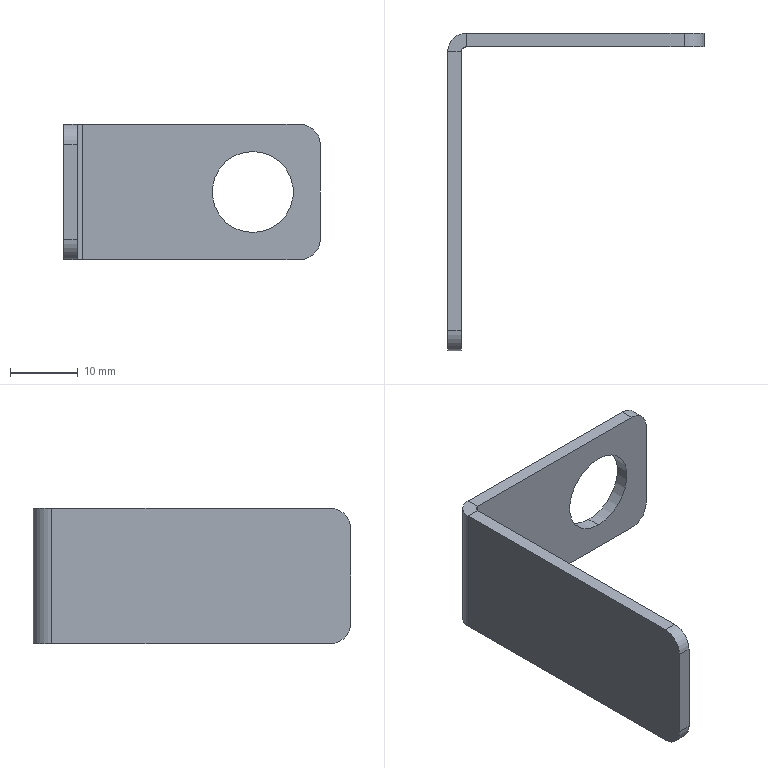Component | SolidWorks | CHEN123-AA-20-1 | 1 solid | 20 faces | box 38 x 47 x 20 mm | volume 3049 mm3 | plane 12 | cylinder 8 | commonest cylinder face diameters 6 x4 12 x2 1.473 x1 5.473 x1
STEP:
#1=CARTESIAN_POINT('',(-0.07876,2.126,-15.984));
#2=VERTEX_POINT('',#1);
#3=CARTESIAN_POINT('',(-0.07876,2.126,-15.512));
#4=VERTEX_POINT('',#3);
#5=CARTESIAN_POINT('',(-0.07876,2.126,-15.748));
#6=DIRECTION('',(-0.,-1.,0.));
#7=DIRECTION('',(-1.,0.,0.));
#8=AXIS2_PLACEMENT_3D('',#5,#6,#7);
#9=CIRCLE('',#8,0.2362);
#10=EDGE_CURVE('',#2,#4,#9,.T.);
#11=ORIENTED_EDGE('',*,*,#10,.T.);
#12=CARTESIAN_POINT('',(-0.07876,2.205,-15.512));
#13=VERTEX_POINT('',#12);
#14=CARTESIAN_POINT('',(-0.07876,2.205,-15.512));
#15=DIRECTION('',(0.,1.,-0.));
#16=VECTOR('',#15,39.37);
#17=LINE('',#14,#16);
#18=EDGE_CURVE('',#4,#13,#17,.T.);
#19=ORIENTED_EDGE('',*,*,#18,.T.);
#20=CARTESIAN_POINT('',(-0.07876,2.205,-15.984));
#21=VERTEX_POINT('',#20);
#22=CARTESIAN_POINT('',(-0.07876,2.205,-15.748));
#23=DIRECTION('',(0.,1.,-0.));
#24=DIRECTION('',(0.,0.,-1.));
#25=AXIS2_PLACEMENT_3D('',#22,#23,#24);
#26=CIRCLE('',#25,0.2362);
#27=EDGE_CURVE('',#13,#21,#26,.T.);
#28=ORIENTED_EDGE('',*,*,#27,.T.);
#29=CARTESIAN_POINT('',(-0.07876,2.205,-15.984));
#30=DIRECTION('',(0.,1.,-0.));
#31=VECTOR('',#30,39.37);
#32=LINE('',#29,#31);
#33=EDGE_CURVE('',#2,#21,#32,.T.);
#34=ORIENTED_EDGE('',*,*,#33,.F.);
#35=EDGE_LOOP('',(#11,#19,#28,#34));
#36=FACE_OUTER_BOUND('',#35,.T.);
#37=CARTESIAN_POINT('',(-0.07876,2.205,-15.748));
#38=DIRECTION('',(0.,1.,-0.));
#39=DIRECTION('',(0.,0.,-1.));
#40=AXIS2_PLACEMENT_3D('',#37,#38,#39);
#41=CYLINDRICAL_SURFACE('',#40,0.2362);
#42=ADVANCED_FACE('',(#36),#41,.F.);
#43=CARTESIAN_POINT('',(-1.073,2.126,-16.142));
#44=VERTEX_POINT('',#43);
#45=CARTESIAN_POINT('',(-1.073,2.205,-16.142));
#46=VERTEX_POINT('',#45);
#47=CARTESIAN_POINT('',(-1.073,2.126,-16.142));
#48=DIRECTION('',(0.,1.,-0.));
#49=VECTOR('',#48,39.37);
#50=LINE('',#47,#49);
#51=EDGE_CURVE('',#44,#46,#50,.T.);
#52=ORIENTED_EDGE('',*,*,#51,.F.);
#53=CARTESIAN_POINT('',(-1.102,2.097,-16.142));
#54=VERTEX_POINT('',#53);
#55=CARTESIAN_POINT('',(-1.073,2.097,-16.142));
#56=DIRECTION('',(0.,-0.,-1.));
#57=DIRECTION('',(1.,0.,0.));
#58=AXIS2_PLACEMENT_3D('',#55,#56,#57);
#59=CIRCLE('',#58,0.029);
#60=EDGE_CURVE('',#54,#44,#59,.T.);
#61=ORIENTED_EDGE('',*,*,#60,.F.);
#62=CARTESIAN_POINT('',(-1.181,2.097,-16.142));
#63=VERTEX_POINT('',#62);
#64=CARTESIAN_POINT('',(-1.181,2.097,-16.142));
#65=DIRECTION('',(1.,0.,-0.));
#66=VECTOR('',#65,39.37);
#67=LINE('',#64,#66);
#68=EDGE_CURVE('',#63,#54,#67,.T.);
#69=ORIENTED_EDGE('',*,*,#68,.F.);
#70=CARTESIAN_POINT('',(-1.073,2.097,-16.142));
#71=DIRECTION('',(0.,-0.,-1.));
#72=DIRECTION('',(-1.,0.,0.));
#73=AXIS2_PLACEMENT_3D('',#70,#71,#72);
#74=CIRCLE('',#73,0.1077);
#75=EDGE_CURVE('',#63,#46,#74,.T.);
#76=ORIENTED_EDGE('',*,*,#75,.T.);
#77=EDGE_LOOP('',(#52,#61,#69,#76));
#78=FACE_OUTER_BOUND('',#77,.T.);
#79=CARTESIAN_POINT('',(-1.073,2.126,-16.142));
#80=DIRECTION('',(0.,-0.,-1.));
#81=DIRECTION('',(-1.,0.,0.));
#82=AXIS2_PLACEMENT_3D('',#79,#80,#81);
#83=PLANE('',#82);
#84=ADVANCED_FACE('',(#78),#83,.T.);
#85=CARTESIAN_POINT('',(0.1968,2.205,-16.142));
#86=VERTEX_POINT('',#85);
#87=CARTESIAN_POINT('',(-1.102,2.205,-16.142));
#88=DIRECTION('',(1.,-0.,0.));
#89=VECTOR('',#88,39.37);
#90=LINE('',#87,#89);
#91=EDGE_CURVE('',#46,#86,#90,.T.);
#92=ORIENTED_EDGE('',*,*,#91,.T.);
#93=CARTESIAN_POINT('',(0.1968,2.126,-16.142));
#94=VERTEX_POINT('',#93);
#95=CARTESIAN_POINT('',(0.1968,2.097,-16.142));
#96=DIRECTION('',(0.,-1.,0.));
#97=VECTOR('',#96,39.37);
#98=LINE('',#95,#97);
#99=EDGE_CURVE('',#86,#94,#98,.T.);
#100=ORIENTED_EDGE('',*,*,#99,.T.);
#101=CARTESIAN_POINT('',(-1.102,2.126,-16.142));
#102=DIRECTION('',(1.,-0.,0.));
#103=VECTOR('',#102,39.37);
#104=LINE('',#101,#103);
#105=EDGE_CURVE('',#44,#94,#104,.T.);
#106=ORIENTED_EDGE('',*,*,#105,.F.);
#107=ORIENTED_EDGE('',*,*,#51,.T.);
#108=EDGE_LOOP('',(#92,#100,#106,#107));
#109=FACE_OUTER_BOUND('',#108,.T.);
#110=CARTESIAN_POINT('',(-1.181,2.097,-16.142));
#111=DIRECTION('',(0.,-0.,-1.));
#112=DIRECTION('',(-1.,0.,0.));
#113=AXIS2_PLACEMENT_3D('',#110,#111,#112);
#114=PLANE('',#113);
#115=ADVANCED_FACE('',(#109),#114,.T.);
#116=CARTESIAN_POINT('',(-1.102,2.097,-15.354));
#117=VERTEX_POINT('',#116);
#118=CARTESIAN_POINT('',(-1.181,2.097,-15.354));
#119=VERTEX_POINT('',#118);
#120=CARTESIAN_POINT('',(-1.102,2.097,-15.354));
#121=DIRECTION('',(-1.,-0.,0.));
#122=VECTOR('',#121,39.37);
#123=LINE('',#120,#122);
#124=EDGE_CURVE('',#117,#119,#123,.T.);
#125=ORIENTED_EDGE('',*,*,#124,.F.);
#126=CARTESIAN_POINT('',(-1.073,2.126,-15.354));
#127=VERTEX_POINT('',#126);
#128=CARTESIAN_POINT('',(-1.073,2.097,-15.354));
#129=DIRECTION('',(0.,-0.,-1.));
#130=DIRECTION('',(1.,0.,0.));
#131=AXIS2_PLACEMENT_3D('',#128,#129,#130);
#132=CIRCLE('',#131,0.029);
#133=EDGE_CURVE('',#117,#127,#132,.T.);
#134=ORIENTED_EDGE('',*,*,#133,.T.);
#135=CARTESIAN_POINT('',(-1.073,2.205,-15.354));
#136=VERTEX_POINT('',#135);
#137=CARTESIAN_POINT('',(-1.073,2.205,-15.354));
#138=DIRECTION('',(-0.,-1.,0.));
#139=VECTOR('',#138,39.37);
#140=LINE('',#137,#139);
#141=EDGE_CURVE('',#136,#127,#140,.T.);
#142=ORIENTED_EDGE('',*,*,#141,.F.);
#143=CARTESIAN_POINT('',(-1.073,2.097,-15.354));
#144=DIRECTION('',(0.,-0.,-1.));
#145=DIRECTION('',(-1.,0.,0.));
#146=AXIS2_PLACEMENT_3D('',#143,#144,#145);
#147=CIRCLE('',#146,0.1077);
#148=EDGE_CURVE('',#119,#136,#147,.T.);
#149=ORIENTED_EDGE('',*,*,#148,.F.);
#150=EDGE_LOOP('',(#125,#134,#142,#149));
#151=FACE_OUTER_BOUND('',#150,.T.);
#152=CARTESIAN_POINT('',(-1.102,2.097,-15.354));
#153=DIRECTION('',(0.,0.,1.));
#154=DIRECTION('',(1.,0.,0.));
#155=AXIS2_PLACEMENT_3D('',#152,#153,#154);
#156=PLANE('',#155);
#157=ADVANCED_FACE('',(#151),#156,.T.);
#158=CARTESIAN_POINT('',(-1.181,0.4725,-15.354));
#159=VERTEX_POINT('',#158);
#160=CARTESIAN_POINT('',(-1.181,0.3544,-15.354));
#161=DIRECTION('',(0.,1.,-0.));
#162=VECTOR('',#161,39.37);
#163=LINE('',#160,#162);
#164=EDGE_CURVE('',#159,#119,#163,.T.);
#165=ORIENTED_EDGE('',*,*,#164,.F.);
#166=CARTESIAN_POINT('',(-1.102,0.4725,-15.354));
#167=VERTEX_POINT('',#166);
#168=CARTESIAN_POINT('',(-1.073,0.4725,-15.354));
#169=DIRECTION('',(1.,0.,0.));
#170=VECTOR('',#169,39.37);
#171=LINE('',#168,#170);
#172=EDGE_CURVE('',#159,#167,#171,.T.);
#173=ORIENTED_EDGE('',*,*,#172,.T.);
#174=CARTESIAN_POINT('',(-1.102,0.3544,-15.354));
#175=DIRECTION('',(0.,1.,-0.));
#176=VECTOR('',#175,39.37);
#177=LINE('',#174,#176);
#178=EDGE_CURVE('',#167,#117,#177,.T.);
#179=ORIENTED_EDGE('',*,*,#178,.T.);
#180=ORIENTED_EDGE('',*,*,#124,.T.);
#181=EDGE_LOOP('',(#165,#173,#179,#180));
#182=FACE_OUTER_BOUND('',#181,.T.);
#183=CARTESIAN_POINT('',(-1.073,2.205,-15.354));
#184=DIRECTION('',(0.,0.,1.));
#185=DIRECTION('',(1.,0.,0.));
#186=AXIS2_PLACEMENT_3D('',#183,#184,#185);
#187=PLANE('',#186);
#188=ADVANCED_FACE('',(#182),#187,.T.);
#189=CARTESIAN_POINT('',(-0.07876,2.205,-15.748));
#190=DIRECTION('',(0.,1.,-0.));
#191=DIRECTION('',(0.,0.,-1.));
#192=AXIS2_PLACEMENT_3D('',#189,#190,#191);
#193=CIRCLE('',#192,0.2362);
#194=EDGE_CURVE('',#21,#13,#193,.T.);
#195=ORIENTED_EDGE('',*,*,#194,.F.);
#196=ORIENTED_EDGE('',*,*,#27,.F.);
#197=EDGE_LOOP('',(#195,#196));
#198=FACE_BOUND('',#197,.T.);
#199=CARTESIAN_POINT('',(0.1968,2.205,-15.354));
#200=VERTEX_POINT('',#199);
#201=CARTESIAN_POINT('',(-1.102,2.205,-15.354));
#202=DIRECTION('',(1.,-0.,0.));
#203=VECTOR('',#202,39.37);
#204=LINE('',#201,#203);
#205=EDGE_CURVE('',#136,#200,#204,.T.);
#206=ORIENTED_EDGE('',*,*,#205,.T.);
#207=CARTESIAN_POINT('',(0.3149,2.205,-15.472));
#208=VERTEX_POINT('',#207);
#209=CARTESIAN_POINT('',(0.1968,2.205,-15.472));
#210=DIRECTION('',(0.,1.,-0.));
#211=DIRECTION('',(-1.,0.,0.));
#212=AXIS2_PLACEMENT_3D('',#209,#210,#211);
#213=CIRCLE('',#212,0.1181);
#214=EDGE_CURVE('',#200,#208,#213,.T.);
#215=ORIENTED_EDGE('',*,*,#214,.T.);
#216=CARTESIAN_POINT('',(0.3149,2.205,-16.024));
#217=VERTEX_POINT('',#216);
#218=CARTESIAN_POINT('',(0.3149,2.205,-16.142));
#219=DIRECTION('',(0.,0.,1.));
#220=VECTOR('',#219,39.37);
#221=LINE('',#218,#220);
#222=EDGE_CURVE('',#217,#208,#221,.T.);
#223=ORIENTED_EDGE('',*,*,#222,.F.);
#224=CARTESIAN_POINT('',(0.1968,2.205,-16.024));
#225=DIRECTION('',(0.,1.,-0.));
#226=DIRECTION('',(-1.,0.,0.));
#227=AXIS2_PLACEMENT_3D('',#224,#225,#226);
#228=CIRCLE('',#227,0.1181);
#229=EDGE_CURVE('',#217,#86,#228,.T.);
#230=ORIENTED_EDGE('',*,*,#229,.T.);
#231=ORIENTED_EDGE('',*,*,#91,.F.);
#232=CARTESIAN_POINT('',(-1.073,2.205,-16.142));
#233=DIRECTION('',(0.,0.,1.));
#234=VECTOR('',#233,39.37);
#235=LINE('',#232,#234);
#236=EDGE_CURVE('',#46,#136,#235,.T.);
#237=ORIENTED_EDGE('',*,*,#236,.T.);
#238=EDGE_LOOP('',(#206,#215,#223,#230,#231,#237));
#239=FACE_OUTER_BOUND('',#238,.T.);
#240=CARTESIAN_POINT('',(-1.102,2.205,-16.142));
#241=DIRECTION('',(-0.,-1.,0.));
#242=DIRECTION('',(-1.,0.,-0.));
#243=AXIS2_PLACEMENT_3D('',#240,#241,#242);
#244=PLANE('',#243);
#245=ADVANCED_FACE('',(#198,#239),#244,.F.);
#246=ORIENTED_EDGE('',*,*,#222,.T.);
#247=CARTESIAN_POINT('',(0.3149,2.126,-15.472));
#248=VERTEX_POINT('',#247);
#249=CARTESIAN_POINT('',(0.3149,2.126,-15.472));
#250=DIRECTION('',(0.,-1.,0.));
#251=VECTOR('',#250,39.37);
#252=LINE('',#249,#251);
#253=EDGE_CURVE('',#208,#248,#252,.T.);
#254=ORIENTED_EDGE('',*,*,#253,.T.);
#255=CARTESIAN_POINT('',(0.3149,2.126,-16.024));
#256=VERTEX_POINT('',#255);
#257=CARTESIAN_POINT('',(0.3149,2.126,-16.142));
#258=DIRECTION('',(0.,0.,1.));
#259=VECTOR('',#258,39.37);
#260=LINE('',#257,#259);
#261=EDGE_CURVE('',#256,#248,#260,.T.);
#262=ORIENTED_EDGE('',*,*,#261,.F.);
#263=CARTESIAN_POINT('',(0.3149,2.126,-16.024));
#264=DIRECTION('',(0.,1.,-0.));
#265=VECTOR('',#264,39.37);
#266=LINE('',#263,#265);
#267=EDGE_CURVE('',#256,#217,#266,.T.);
#268=ORIENTED_EDGE('',*,*,#267,.T.);
#269=EDGE_LOOP('',(#246,#254,#262,#268));
#270=FACE_OUTER_BOUND('',#269,.T.);
#271=CARTESIAN_POINT('',(0.3149,2.126,-16.142));
#272=DIRECTION('',(1.,0.,0.));
#273=DIRECTION('',(0.,-0.,-1.));
#274=AXIS2_PLACEMENT_3D('',#271,#272,#273);
#275=PLANE('',#274);
#276=ADVANCED_FACE('',(#270),#275,.T.);
#277=ORIENTED_EDGE('',*,*,#10,.F.);
#278=CARTESIAN_POINT('',(-0.07876,2.126,-15.748));
#279=DIRECTION('',(-0.,-1.,0.));
#280=DIRECTION('',(-1.,0.,0.));
#281=AXIS2_PLACEMENT_3D('',#278,#279,#280);
#282=CIRCLE('',#281,0.2362);
#283=EDGE_CURVE('',#4,#2,#282,.T.);
#284=ORIENTED_EDGE('',*,*,#283,.F.);
#285=EDGE_LOOP('',(#277,#284));
#286=FACE_BOUND('',#285,.T.);
#287=ORIENTED_EDGE('',*,*,#261,.T.);
#288=CARTESIAN_POINT('',(0.1968,2.126,-15.354));
#289=VERTEX_POINT('',#288);
#290=CARTESIAN_POINT('',(0.1968,2.126,-15.472));
#291=DIRECTION('',(-0.,-1.,0.));
#292=DIRECTION('',(-1.,0.,0.));
#293=AXIS2_PLACEMENT_3D('',#290,#291,#292);
#294=CIRCLE('',#293,0.1181);
#295=EDGE_CURVE('',#248,#289,#294,.T.);
#296=ORIENTED_EDGE('',*,*,#295,.T.);
#297=CARTESIAN_POINT('',(-1.102,2.126,-15.354));
#298=DIRECTION('',(1.,-0.,0.));
#299=VECTOR('',#298,39.37);
#300=LINE('',#297,#299);
#301=EDGE_CURVE('',#127,#289,#300,.T.);
#302=ORIENTED_EDGE('',*,*,#301,.F.);
#303=CARTESIAN_POINT('',(-1.073,2.126,-16.142));
#304=DIRECTION('',(0.,0.,1.));
#305=VECTOR('',#304,39.37);
#306=LINE('',#303,#305);
#307=EDGE_CURVE('',#44,#127,#306,.T.);
#308=ORIENTED_EDGE('',*,*,#307,.F.);
#309=ORIENTED_EDGE('',*,*,#105,.T.);
#310=CARTESIAN_POINT('',(0.1968,2.126,-16.024));
#311=DIRECTION('',(-0.,-1.,0.));
#312=DIRECTION('',(-1.,0.,0.));
#313=AXIS2_PLACEMENT_3D('',#310,#311,#312);
#314=CIRCLE('',#313,0.1181);
#315=EDGE_CURVE('',#94,#256,#314,.T.);
#316=ORIENTED_EDGE('',*,*,#315,.T.);
#317=EDGE_LOOP('',(#287,#296,#302,#308,#309,#316));
#318=FACE_OUTER_BOUND('',#317,.T.);
#319=CARTESIAN_POINT('',(-1.102,2.126,-16.142));
#320=DIRECTION('',(-0.,-1.,0.));
#321=DIRECTION('',(-1.,0.,-0.));
#322=AXIS2_PLACEMENT_3D('',#319,#320,#321);
#323=PLANE('',#322);
#324=ADVANCED_FACE('',(#286,#318),#323,.T.);
#325=ORIENTED_EDGE('',*,*,#133,.F.);
#326=CARTESIAN_POINT('',(-1.102,2.097,-16.142));
#327=DIRECTION('',(0.,0.,1.));
#328=VECTOR('',#327,39.37);
#329=LINE('',#326,#328);
#330=EDGE_CURVE('',#54,#117,#329,.T.);
#331=ORIENTED_EDGE('',*,*,#330,.F.);
#332=ORIENTED_EDGE('',*,*,#60,.T.);
#333=ORIENTED_EDGE('',*,*,#307,.T.);
#334=EDGE_LOOP('',(#325,#331,#332,#333));
#335=FACE_OUTER_BOUND('',#334,.T.);
#336=CARTESIAN_POINT('',(-1.073,2.097,-16.142));
#337=DIRECTION('',(0.,0.,1.));
#338=DIRECTION('',(1.,0.,0.));
#339=AXIS2_PLACEMENT_3D('',#336,#337,#338);
#340=CYLINDRICAL_SURFACE('',#339,0.029);
#341=ADVANCED_FACE('',(#335),#340,.F.);
#342=ORIENTED_EDGE('',*,*,#178,.F.);
#343=CARTESIAN_POINT('',(-1.102,0.3544,-15.472));
#344=VERTEX_POINT('',#343);
#345=CARTESIAN_POINT('',(-1.102,0.4725,-15.472));
#346=DIRECTION('',(1.,0.,0.));
#347=DIRECTION('',(0.,0.,-1.));
#348=AXIS2_PLACEMENT_3D('',#345,#346,#347);
#349=CIRCLE('',#348,0.1181);
#350=EDGE_CURVE('',#167,#344,#349,.T.);
#351=ORIENTED_EDGE('',*,*,#350,.T.);
#352=CARTESIAN_POINT('',(-1.102,0.3544,-16.024));
#353=VERTEX_POINT('',#352);
#354=CARTESIAN_POINT('',(-1.102,0.3544,-16.142));
#355=DIRECTION('',(0.,0.,1.));
#356=VECTOR('',#355,39.37);
#357=LINE('',#354,#356);
#358=EDGE_CURVE('',#353,#344,#357,.T.);
#359=ORIENTED_EDGE('',*,*,#358,.F.);
#360=CARTESIAN_POINT('',(-1.102,0.4725,-16.142));
#361=VERTEX_POINT('',#360);
#362=CARTESIAN_POINT('',(-1.102,0.4725,-16.024));
#363=DIRECTION('',(1.,0.,0.));
#364=DIRECTION('',(0.,0.,-1.));
#365=AXIS2_PLACEMENT_3D('',#362,#363,#364);
#366=CIRCLE('',#365,0.1181);
#367=EDGE_CURVE('',#353,#361,#366,.T.);
#368=ORIENTED_EDGE('',*,*,#367,.T.);
#369=CARTESIAN_POINT('',(-1.102,0.3544,-16.142));
#370=DIRECTION('',(0.,1.,-0.));
#371=VECTOR('',#370,39.37);
#372=LINE('',#369,#371);
#373=EDGE_CURVE('',#361,#54,#372,.T.);
#374=ORIENTED_EDGE('',*,*,#373,.T.);
#375=ORIENTED_EDGE('',*,*,#330,.T.);
#376=EDGE_LOOP('',(#342,#351,#359,#368,#374,#375));
#377=FACE_OUTER_BOUND('',#376,.T.);
#378=CARTESIAN_POINT('',(-1.102,0.3544,-16.142));
#379=DIRECTION('',(1.,0.,0.));
#380=DIRECTION('',(0.,-0.,-1.));
#381=AXIS2_PLACEMENT_3D('',#378,#379,#380);
#382=PLANE('',#381);
#383=ADVANCED_FACE('',(#377),#382,.T.);
#384=ORIENTED_EDGE('',*,*,#358,.T.);
#385=CARTESIAN_POINT('',(-1.181,0.3544,-15.472));
#386=VERTEX_POINT('',#385);
#387=CARTESIAN_POINT('',(-1.181,0.3544,-15.472));
#388=DIRECTION('',(-1.,0.,0.));
#389=VECTOR('',#388,39.37);
#390=LINE('',#387,#389);
#391=EDGE_CURVE('',#344,#386,#390,.T.);
#392=ORIENTED_EDGE('',*,*,#391,.T.);
#393=CARTESIAN_POINT('',(-1.181,0.3544,-16.024));
#394=VERTEX_POINT('',#393);
#395=CARTESIAN_POINT('',(-1.181,0.3544,-16.142));
#396=DIRECTION('',(0.,0.,1.));
#397=VECTOR('',#396,39.37);
#398=LINE('',#395,#397);
#399=EDGE_CURVE('',#394,#386,#398,.T.);
#400=ORIENTED_EDGE('',*,*,#399,.F.);
#401=CARTESIAN_POINT('',(-1.102,0.3544,-16.024));
#402=DIRECTION('',(1.,0.,0.));
#403=VECTOR('',#402,39.37);
#404=LINE('',#401,#403);
#405=EDGE_CURVE('',#394,#353,#404,.T.);
#406=ORIENTED_EDGE('',*,*,#405,.T.);
#407=EDGE_LOOP('',(#384,#392,#400,#406));
#408=FACE_OUTER_BOUND('',#407,.T.);
#409=CARTESIAN_POINT('',(-1.181,0.3544,-16.142));
#410=DIRECTION('',(0.,-1.,0.));
#411=DIRECTION('',(0.,0.,1.));
#412=AXIS2_PLACEMENT_3D('',#409,#410,#411);
#413=PLANE('',#412);
#414=ADVANCED_FACE('',(#408),#413,.T.);
#415=ORIENTED_EDGE('',*,*,#399,.T.);
#416=CARTESIAN_POINT('',(-1.181,0.4725,-15.472));
#417=DIRECTION('',(-1.,0.,0.));
#418=DIRECTION('',(0.,0.,-1.));
#419=AXIS2_PLACEMENT_3D('',#416,#417,#418);
#420=CIRCLE('',#419,0.1181);
#421=EDGE_CURVE('',#386,#159,#420,.T.);
#422=ORIENTED_EDGE('',*,*,#421,.T.);
#423=ORIENTED_EDGE('',*,*,#164,.T.);
#424=CARTESIAN_POINT('',(-1.181,2.097,-16.142));
#425=DIRECTION('',(0.,0.,1.));
#426=VECTOR('',#425,39.37);
#427=LINE('',#424,#426);
#428=EDGE_CURVE('',#63,#119,#427,.T.);
#429=ORIENTED_EDGE('',*,*,#428,.F.);
#430=CARTESIAN_POINT('',(-1.181,0.4725,-16.142));
#431=VERTEX_POINT('',#430);
#432=CARTESIAN_POINT('',(-1.181,0.3544,-16.142));
#433=DIRECTION('',(0.,1.,-0.));
#434=VECTOR('',#433,39.37);
#435=LINE('',#432,#434);
#436=EDGE_CURVE('',#431,#63,#435,.T.);
#437=ORIENTED_EDGE('',*,*,#436,.F.);
#438=CARTESIAN_POINT('',(-1.181,0.4725,-16.024));
#439=DIRECTION('',(-1.,0.,0.));
#440=DIRECTION('',(0.,0.,-1.));
#441=AXIS2_PLACEMENT_3D('',#438,#439,#440);
#442=CIRCLE('',#441,0.1181);
#443=EDGE_CURVE('',#431,#394,#442,.T.);
#444=ORIENTED_EDGE('',*,*,#443,.T.);
#445=EDGE_LOOP('',(#415,#422,#423,#429,#437,#444));
#446=FACE_OUTER_BOUND('',#445,.T.);
#447=CARTESIAN_POINT('',(-1.181,0.3544,-16.142));
#448=DIRECTION('',(1.,0.,0.));
#449=DIRECTION('',(0.,-0.,-1.));
#450=AXIS2_PLACEMENT_3D('',#447,#448,#449);
#451=PLANE('',#450);
#452=ADVANCED_FACE('',(#446),#451,.F.);
#453=ORIENTED_EDGE('',*,*,#148,.T.);
#454=ORIENTED_EDGE('',*,*,#236,.F.);
#455=ORIENTED_EDGE('',*,*,#75,.F.);
#456=ORIENTED_EDGE('',*,*,#428,.T.);
#457=EDGE_LOOP('',(#453,#454,#455,#456));
#458=FACE_OUTER_BOUND('',#457,.T.);
#459=CARTESIAN_POINT('',(-1.073,2.097,-16.142));
#460=DIRECTION('',(0.,0.,1.));
#461=DIRECTION('',(1.,0.,0.));
#462=AXIS2_PLACEMENT_3D('',#459,#460,#461);
#463=CYLINDRICAL_SURFACE('',#462,0.1077);
#464=ADVANCED_FACE('',(#458),#463,.T.);
#465=ORIENTED_EDGE('',*,*,#373,.F.);
#466=CARTESIAN_POINT('',(-1.181,0.4725,-16.142));
#467=DIRECTION('',(-1.,0.,0.));
#468=VECTOR('',#467,39.37);
#469=LINE('',#466,#468);
#470=EDGE_CURVE('',#361,#431,#469,.T.);
#471=ORIENTED_EDGE('',*,*,#470,.T.);
#472=ORIENTED_EDGE('',*,*,#436,.T.);
#473=ORIENTED_EDGE('',*,*,#68,.T.);
#474=EDGE_LOOP('',(#465,#471,#472,#473));
#475=FACE_OUTER_BOUND('',#474,.T.);
#476=CARTESIAN_POINT('',(-1.073,2.097,-16.142));
#477=DIRECTION('',(0.,0.,1.));
#478=DIRECTION('',(1.,0.,0.));
#479=AXIS2_PLACEMENT_3D('',#476,#477,#478);
#480=PLANE('',#479);
#481=ADVANCED_FACE('',(#475),#480,.F.);
#482=ORIENTED_EDGE('',*,*,#301,.T.);
#483=CARTESIAN_POINT('',(0.1968,2.097,-15.354));
#484=DIRECTION('',(0.,1.,-0.));
#485=VECTOR('',#484,39.37);
#486=LINE('',#483,#485);
#487=EDGE_CURVE('',#289,#200,#486,.T.);
#488=ORIENTED_EDGE('',*,*,#487,.T.);
#489=ORIENTED_EDGE('',*,*,#205,.F.);
#490=ORIENTED_EDGE('',*,*,#141,.T.);
#491=EDGE_LOOP('',(#482,#488,#489,#490));
#492=FACE_OUTER_BOUND('',#491,.T.);
#493=CARTESIAN_POINT('',(-1.073,2.097,-15.354));
#494=DIRECTION('',(0.,0.,1.));
#495=DIRECTION('',(1.,0.,0.));
#496=AXIS2_PLACEMENT_3D('',#493,#494,#495);
#497=PLANE('',#496);
#498=ADVANCED_FACE('',(#492),#497,.T.);
#499=ORIENTED_EDGE('',*,*,#18,.F.);
#500=ORIENTED_EDGE('',*,*,#283,.T.);
#501=ORIENTED_EDGE('',*,*,#33,.T.);
#502=ORIENTED_EDGE('',*,*,#194,.T.);
#503=EDGE_LOOP('',(#499,#500,#501,#502));
#504=FACE_OUTER_BOUND('',#503,.T.);
#505=CARTESIAN_POINT('',(-0.07876,2.205,-15.748));
#506=DIRECTION('',(0.,1.,-0.));
#507=DIRECTION('',(0.,0.,-1.));
#508=AXIS2_PLACEMENT_3D('',#505,#506,#507);
#509=CYLINDRICAL_SURFACE('',#508,0.2362);
#510=ADVANCED_FACE('',(#504),#509,.F.);
#511=ORIENTED_EDGE('',*,*,#421,.F.);
#512=ORIENTED_EDGE('',*,*,#391,.F.);
#513=ORIENTED_EDGE('',*,*,#350,.F.);
#514=ORIENTED_EDGE('',*,*,#172,.F.);
#515=EDGE_LOOP('',(#511,#512,#513,#514));
#516=FACE_OUTER_BOUND('',#515,.T.);
#517=CARTESIAN_POINT('',(-1.073,0.4725,-15.472));
#518=DIRECTION('',(1.,0.,0.));
#519=DIRECTION('',(0.,0.,-1.));
#520=AXIS2_PLACEMENT_3D('',#517,#518,#519);
#521=CYLINDRICAL_SURFACE('',#520,0.1181);
#522=ADVANCED_FACE('',(#516),#521,.T.);
#523=ORIENTED_EDGE('',*,*,#443,.F.);
#524=ORIENTED_EDGE('',*,*,#470,.F.);
#525=ORIENTED_EDGE('',*,*,#367,.F.);
#526=ORIENTED_EDGE('',*,*,#405,.F.);
#527=EDGE_LOOP('',(#523,#524,#525,#526));
#528=FACE_OUTER_BOUND('',#527,.T.);
#529=CARTESIAN_POINT('',(-1.181,0.4725,-16.024));
#530=DIRECTION('',(-1.,0.,0.));
#531=DIRECTION('',(0.,0.,1.));
#532=AXIS2_PLACEMENT_3D('',#529,#530,#531);
#533=CYLINDRICAL_SURFACE('',#532,0.1181);
#534=ADVANCED_FACE('',(#528),#533,.T.);
#535=ORIENTED_EDGE('',*,*,#295,.F.);
#536=ORIENTED_EDGE('',*,*,#253,.F.);
#537=ORIENTED_EDGE('',*,*,#214,.F.);
#538=ORIENTED_EDGE('',*,*,#487,.F.);
#539=EDGE_LOOP('',(#535,#536,#537,#538));
#540=FACE_OUTER_BOUND('',#539,.T.);
#541=CARTESIAN_POINT('',(0.1968,2.097,-15.472));
#542=DIRECTION('',(0.,1.,-0.));
#543=DIRECTION('',(0.,0.,-1.));
#544=AXIS2_PLACEMENT_3D('',#541,#542,#543);
#545=CYLINDRICAL_SURFACE('',#544,0.1181);
#546=ADVANCED_FACE('',(#540),#545,.T.);
#547=ORIENTED_EDGE('',*,*,#315,.F.);
#548=ORIENTED_EDGE('',*,*,#99,.F.);
#549=ORIENTED_EDGE('',*,*,#229,.F.);
#550=ORIENTED_EDGE('',*,*,#267,.F.);
#551=EDGE_LOOP('',(#547,#548,#549,#550));
#552=FACE_OUTER_BOUND('',#551,.T.);
#553=CARTESIAN_POINT('',(0.1968,2.126,-16.024));
#554=DIRECTION('',(0.,1.,-0.));
#555=DIRECTION('',(0.,0.,-1.));
#556=AXIS2_PLACEMENT_3D('',#553,#554,#555);
#557=CYLINDRICAL_SURFACE('',#556,0.1181);
#558=ADVANCED_FACE('',(#552),#557,.T.);
#559=CLOSED_SHELL('',(#42,#84,#115,#157,#188,#245,#276,#324,#341,#383,#414,#452,#464,#481,#498,#510,#522,#534,#546,#558));
#560=MANIFOLD_SOLID_BREP('',#559);
#561=CARTESIAN_POINT('',(0.,0.,0.));
#562=DIRECTION('',(0.,0.,1.));
#563=DIRECTION('',(1.,0.,0.));
#564=AXIS2_PLACEMENT_3D('',#561,#562,#563);
#565=(LENGTH_UNIT()NAMED_UNIT(*)SI_UNIT($,.METRE.));
#566=LENGTH_MEASURE_WITH_UNIT(LENGTH_MEASURE(0.0254),#565);
#567=DIMENSIONAL_EXPONENTS(1.,0.,0.,0.,0.,0.,0.);
#568=(CONVERSION_BASED_UNIT('',#566)LENGTH_UNIT()NAMED_UNIT(#567));
#569=UNCERTAINTY_MEASURE_WITH_UNIT(LENGTH_MEASURE(0.00001),#568,'','');
#570=(NAMED_UNIT(*)PLANE_ANGLE_UNIT()SI_UNIT($,.RADIAN.));
#571=(NAMED_UNIT(*)SI_UNIT($,.STERADIAN.)SOLID_ANGLE_UNIT());
#572=(GEOMETRIC_REPRESENTATION_CONTEXT(3)GLOBAL_UNCERTAINTY_ASSIGNED_CONTEXT((#569))GLOBAL_UNIT_ASSIGNED_CONTEXT((#568,#570,#571))REPRESENTATION_CONTEXT('',''));
#573=ADVANCED_BREP_SHAPE_REPRESENTATION('',(#560,#564),#572);
#574=COLOUR_RGB('',0.7922,0.8196,0.9333);
#575=FILL_AREA_STYLE_COLOUR('',#574);
#576=FILL_AREA_STYLE('',(#575));
#577=SURFACE_STYLE_FILL_AREA(#576);
#578=SURFACE_SIDE_STYLE('',(#577));
#579=SURFACE_STYLE_USAGE(.BOTH.,#578);
#580=PRESENTATION_STYLE_ASSIGNMENT((#579));
#581=STYLED_ITEM('',(#580),#560);
#582=(LENGTH_UNIT()NAMED_UNIT(*)SI_UNIT($,.METRE.));
#583=LENGTH_MEASURE_WITH_UNIT(LENGTH_MEASURE(0.0254),#582);
#584=DIMENSIONAL_EXPONENTS(1.,0.,0.,0.,0.,0.,0.);
#585=(CONVERSION_BASED_UNIT('',#583)LENGTH_UNIT()NAMED_UNIT(#584));
#586=UNCERTAINTY_MEASURE_WITH_UNIT(LENGTH_MEASURE(0.00001),#585,'','');
#587=(NAMED_UNIT(*)PLANE_ANGLE_UNIT()SI_UNIT($,.RADIAN.));
#588=(NAMED_UNIT(*)SI_UNIT($,.STERADIAN.)SOLID_ANGLE_UNIT());
#589=(GEOMETRIC_REPRESENTATION_CONTEXT(3)GLOBAL_UNCERTAINTY_ASSIGNED_CONTEXT((#586))GLOBAL_UNIT_ASSIGNED_CONTEXT((#585,#587,#588))REPRESENTATION_CONTEXT('',''));
#590=MECHANICAL_DESIGN_GEOMETRIC_PRESENTATION_REPRESENTATION('',(#581),#589);
#591=PRESENTATION_LAYER_ASSIGNMENT('','',(#581));